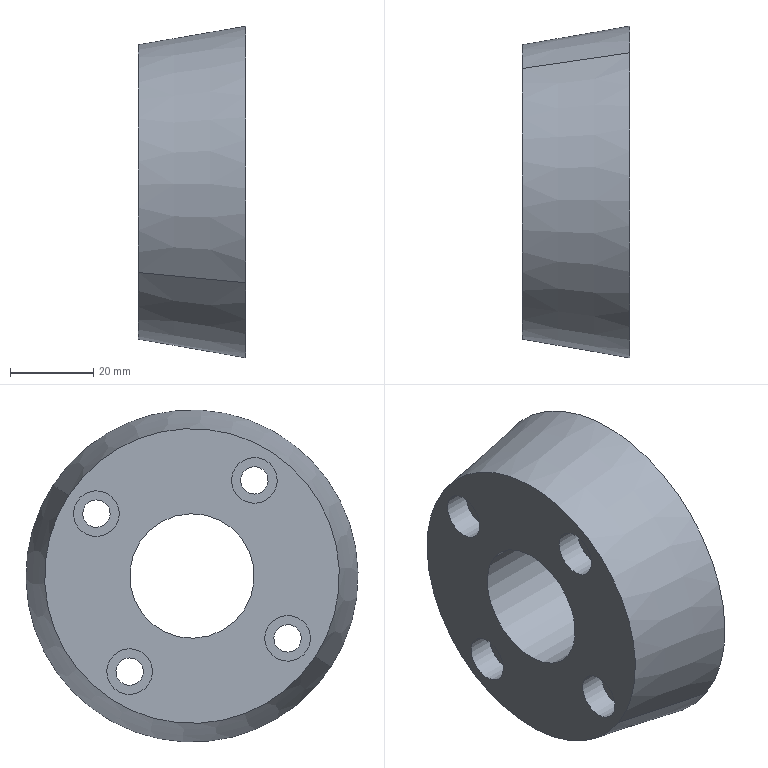Component | SolidWorks | LocatingSleeve3-1_LocatingSleeve3-2-1 | 1 solid | 26 faces | box 26 x 80 x 80 mm | volume 93046 mm3 | cylinder 18 | plane 6 | cone 2 | commonest cylinder face diameters 11 x8 6.6 x8 30 x2
STEP:
#1=CARTESIAN_POINT('',(12.546,-0.9808,30.92));
#2=VERTEX_POINT('',#1);
#3=CARTESIAN_POINT('',(12.546,-0.6181,31.156));
#4=VERTEX_POINT('',#3);
#5=CARTESIAN_POINT('',(12.546,-0.7995,31.038));
#6=DIRECTION('',(-1.,-0.,0.));
#7=DIRECTION('',(0.,0.8375,0.5465));
#8=AXIS2_PLACEMENT_3D('',#5,#6,#7);
#9=CIRCLE('',#8,0.2165);
#10=EDGE_CURVE('',#2,#4,#9,.T.);
#11=ORIENTED_EDGE('',*,*,#10,.F.);
#12=CARTESIAN_POINT('',(12.294,-0.9808,30.92));
#13=VERTEX_POINT('',#12);
#14=CARTESIAN_POINT('',(12.294,-0.9808,30.92));
#15=DIRECTION('',(-1.,-0.,0.));
#16=VECTOR('',#15,39.37);
#17=LINE('',#14,#16);
#18=EDGE_CURVE('',#2,#13,#17,.T.);
#19=ORIENTED_EDGE('',*,*,#18,.T.);
#20=CARTESIAN_POINT('',(12.294,-0.6181,31.156));
#21=VERTEX_POINT('',#20);
#22=CARTESIAN_POINT('',(12.294,-0.7995,31.038));
#23=DIRECTION('',(-1.,-0.,0.));
#24=DIRECTION('',(0.,0.8375,0.5465));
#25=AXIS2_PLACEMENT_3D('',#22,#23,#24);
#26=CIRCLE('',#25,0.2165);
#27=EDGE_CURVE('',#13,#21,#26,.T.);
#28=ORIENTED_EDGE('',*,*,#27,.T.);
#29=CARTESIAN_POINT('',(12.294,-0.6181,31.156));
#30=DIRECTION('',(-1.,-0.,0.));
#31=VECTOR('',#30,39.37);
#32=LINE('',#29,#31);
#33=EDGE_CURVE('',#4,#21,#32,.T.);
#34=ORIENTED_EDGE('',*,*,#33,.F.);
#35=EDGE_LOOP('',(#11,#19,#28,#34));
#36=FACE_OUTER_BOUND('',#35,.T.);
#37=CARTESIAN_POINT('',(12.294,-0.7995,31.038));
#38=DIRECTION('',(-1.,-0.,0.));
#39=DIRECTION('',(0.,0.8375,0.5465));
#40=AXIS2_PLACEMENT_3D('',#37,#38,#39);
#41=CYLINDRICAL_SURFACE('',#40,0.2165);
#42=ADVANCED_FACE('',(#36),#41,.F.);
#43=CARTESIAN_POINT('',(13.318,-0.9083,30.967));
#44=VERTEX_POINT('',#43);
#45=CARTESIAN_POINT('',(13.318,-0.6907,31.109));
#46=VERTEX_POINT('',#45);
#47=CARTESIAN_POINT('',(13.318,-0.7995,31.038));
#48=DIRECTION('',(-1.,-0.,0.));
#49=DIRECTION('',(0.,0.8375,0.5465));
#50=AXIS2_PLACEMENT_3D('',#47,#48,#49);
#51=CIRCLE('',#50,0.1299);
#52=EDGE_CURVE('',#44,#46,#51,.T.);
#53=ORIENTED_EDGE('',*,*,#52,.F.);
#54=CARTESIAN_POINT('',(12.546,-0.9083,30.967));
#55=VERTEX_POINT('',#54);
#56=CARTESIAN_POINT('',(12.294,-0.9083,30.967));
#57=DIRECTION('',(-1.,-0.,0.));
#58=VECTOR('',#57,39.37);
#59=LINE('',#56,#58);
#60=EDGE_CURVE('',#44,#55,#59,.T.);
#61=ORIENTED_EDGE('',*,*,#60,.T.);
#62=CARTESIAN_POINT('',(12.546,-0.6907,31.109));
#63=VERTEX_POINT('',#62);
#64=CARTESIAN_POINT('',(12.546,-0.7995,31.038));
#65=DIRECTION('',(-1.,-0.,0.));
#66=DIRECTION('',(0.,0.8375,0.5465));
#67=AXIS2_PLACEMENT_3D('',#64,#65,#66);
#68=CIRCLE('',#67,0.1299);
#69=EDGE_CURVE('',#55,#63,#68,.T.);
#70=ORIENTED_EDGE('',*,*,#69,.T.);
#71=CARTESIAN_POINT('',(12.294,-0.6907,31.109));
#72=DIRECTION('',(-1.,-0.,0.));
#73=VECTOR('',#72,39.37);
#74=LINE('',#71,#73);
#75=EDGE_CURVE('',#46,#63,#74,.T.);
#76=ORIENTED_EDGE('',*,*,#75,.F.);
#77=EDGE_LOOP('',(#53,#61,#70,#76));
#78=FACE_OUTER_BOUND('',#77,.T.);
#79=CARTESIAN_POINT('',(12.294,-0.7995,31.038));
#80=DIRECTION('',(-1.,-0.,0.));
#81=DIRECTION('',(0.,0.8375,0.5465));
#82=AXIS2_PLACEMENT_3D('',#79,#80,#81);
#83=CYLINDRICAL_SURFACE('',#82,0.1299);
#84=ADVANCED_FACE('',(#78),#83,.F.);
#85=CARTESIAN_POINT('',(12.546,-0.6657,32.418));
#86=VERTEX_POINT('',#85);
#87=CARTESIAN_POINT('',(12.546,-0.303,32.655));
#88=VERTEX_POINT('',#87);
#89=CARTESIAN_POINT('',(12.546,-0.4844,32.536));
#90=DIRECTION('',(-1.,-0.,0.));
#91=DIRECTION('',(0.,0.8375,0.5465));
#92=AXIS2_PLACEMENT_3D('',#89,#90,#91);
#93=CIRCLE('',#92,0.2165);
#94=EDGE_CURVE('',#86,#88,#93,.T.);
#95=ORIENTED_EDGE('',*,*,#94,.F.);
#96=CARTESIAN_POINT('',(12.294,-0.6657,32.418));
#97=VERTEX_POINT('',#96);
#98=CARTESIAN_POINT('',(12.294,-0.6657,32.418));
#99=DIRECTION('',(-1.,-0.,0.));
#100=VECTOR('',#99,39.37);
#101=LINE('',#98,#100);
#102=EDGE_CURVE('',#86,#97,#101,.T.);
#103=ORIENTED_EDGE('',*,*,#102,.T.);
#104=CARTESIAN_POINT('',(12.294,-0.303,32.655));
#105=VERTEX_POINT('',#104);
#106=CARTESIAN_POINT('',(12.294,-0.4844,32.536));
#107=DIRECTION('',(-1.,-0.,0.));
#108=DIRECTION('',(0.,0.8375,0.5465));
#109=AXIS2_PLACEMENT_3D('',#106,#107,#108);
#110=CIRCLE('',#109,0.2165);
#111=EDGE_CURVE('',#97,#105,#110,.T.);
#112=ORIENTED_EDGE('',*,*,#111,.T.);
#113=CARTESIAN_POINT('',(12.294,-0.303,32.655));
#114=DIRECTION('',(-1.,-0.,0.));
#115=VECTOR('',#114,39.37);
#116=LINE('',#113,#115);
#117=EDGE_CURVE('',#88,#105,#116,.T.);
#118=ORIENTED_EDGE('',*,*,#117,.F.);
#119=EDGE_LOOP('',(#95,#103,#112,#118));
#120=FACE_OUTER_BOUND('',#119,.T.);
#121=CARTESIAN_POINT('',(12.294,-0.4844,32.536));
#122=DIRECTION('',(-1.,-0.,0.));
#123=DIRECTION('',(0.,0.8375,0.5465));
#124=AXIS2_PLACEMENT_3D('',#121,#122,#123);
#125=CYLINDRICAL_SURFACE('',#124,0.2165);
#126=ADVANCED_FACE('',(#120),#125,.F.);
#127=CARTESIAN_POINT('',(13.318,-0.5932,32.465));
#128=VERTEX_POINT('',#127);
#129=CARTESIAN_POINT('',(13.318,-0.3756,32.607));
#130=VERTEX_POINT('',#129);
#131=CARTESIAN_POINT('',(13.318,-0.4844,32.536));
#132=DIRECTION('',(-1.,-0.,0.));
#133=DIRECTION('',(0.,0.8375,0.5465));
#134=AXIS2_PLACEMENT_3D('',#131,#132,#133);
#135=CIRCLE('',#134,0.1299);
#136=EDGE_CURVE('',#128,#130,#135,.T.);
#137=ORIENTED_EDGE('',*,*,#136,.F.);
#138=CARTESIAN_POINT('',(12.546,-0.5932,32.465));
#139=VERTEX_POINT('',#138);
#140=CARTESIAN_POINT('',(12.294,-0.5932,32.465));
#141=DIRECTION('',(-1.,-0.,0.));
#142=VECTOR('',#141,39.37);
#143=LINE('',#140,#142);
#144=EDGE_CURVE('',#128,#139,#143,.T.);
#145=ORIENTED_EDGE('',*,*,#144,.T.);
#146=CARTESIAN_POINT('',(12.546,-0.3756,32.607));
#147=VERTEX_POINT('',#146);
#148=CARTESIAN_POINT('',(12.546,-0.4844,32.536));
#149=DIRECTION('',(-1.,-0.,0.));
#150=DIRECTION('',(0.,0.8375,0.5465));
#151=AXIS2_PLACEMENT_3D('',#148,#149,#150);
#152=CIRCLE('',#151,0.1299);
#153=EDGE_CURVE('',#139,#147,#152,.T.);
#154=ORIENTED_EDGE('',*,*,#153,.T.);
#155=CARTESIAN_POINT('',(12.294,-0.3756,32.607));
#156=DIRECTION('',(-1.,-0.,0.));
#157=VECTOR('',#156,39.37);
#158=LINE('',#155,#157);
#159=EDGE_CURVE('',#130,#147,#158,.T.);
#160=ORIENTED_EDGE('',*,*,#159,.F.);
#161=EDGE_LOOP('',(#137,#145,#154,#160));
#162=FACE_OUTER_BOUND('',#161,.T.);
#163=CARTESIAN_POINT('',(12.294,-0.4844,32.536));
#164=DIRECTION('',(-1.,-0.,0.));
#165=DIRECTION('',(0.,0.8375,0.5465));
#166=AXIS2_PLACEMENT_3D('',#163,#164,#165);
#167=CYLINDRICAL_SURFACE('',#166,0.1299);
#168=ADVANCED_FACE('',(#162),#167,.F.);
#169=CARTESIAN_POINT('',(12.546,-2.164,32.733));
#170=VERTEX_POINT('',#169);
#171=CARTESIAN_POINT('',(12.546,-1.801,32.97));
#172=VERTEX_POINT('',#171);
#173=CARTESIAN_POINT('',(12.546,-1.983,32.852));
#174=DIRECTION('',(-1.,-0.,0.));
#175=DIRECTION('',(0.,0.8375,0.5465));
#176=AXIS2_PLACEMENT_3D('',#173,#174,#175);
#177=CIRCLE('',#176,0.2165);
#178=EDGE_CURVE('',#170,#172,#177,.T.);
#179=ORIENTED_EDGE('',*,*,#178,.F.);
#180=CARTESIAN_POINT('',(12.294,-2.164,32.733));
#181=VERTEX_POINT('',#180);
#182=CARTESIAN_POINT('',(12.294,-2.164,32.733));
#183=DIRECTION('',(-1.,-0.,0.));
#184=VECTOR('',#183,39.37);
#185=LINE('',#182,#184);
#186=EDGE_CURVE('',#170,#181,#185,.T.);
#187=ORIENTED_EDGE('',*,*,#186,.T.);
#188=CARTESIAN_POINT('',(12.294,-1.801,32.97));
#189=VERTEX_POINT('',#188);
#190=CARTESIAN_POINT('',(12.294,-1.983,32.852));
#191=DIRECTION('',(-1.,-0.,0.));
#192=DIRECTION('',(0.,0.8375,0.5465));
#193=AXIS2_PLACEMENT_3D('',#190,#191,#192);
#194=CIRCLE('',#193,0.2165);
#195=EDGE_CURVE('',#181,#189,#194,.T.);
#196=ORIENTED_EDGE('',*,*,#195,.T.);
#197=CARTESIAN_POINT('',(12.294,-1.801,32.97));
#198=DIRECTION('',(-1.,-0.,0.));
#199=VECTOR('',#198,39.37);
#200=LINE('',#197,#199);
#201=EDGE_CURVE('',#172,#189,#200,.T.);
#202=ORIENTED_EDGE('',*,*,#201,.F.);
#203=EDGE_LOOP('',(#179,#187,#196,#202));
#204=FACE_OUTER_BOUND('',#203,.T.);
#205=CARTESIAN_POINT('',(12.294,-1.983,32.852));
#206=DIRECTION('',(-1.,-0.,0.));
#207=DIRECTION('',(0.,0.8375,0.5465));
#208=AXIS2_PLACEMENT_3D('',#205,#206,#207);
#209=CYLINDRICAL_SURFACE('',#208,0.2165);
#210=ADVANCED_FACE('',(#204),#209,.F.);
#211=CARTESIAN_POINT('',(13.318,-2.092,32.781));
#212=VERTEX_POINT('',#211);
#213=CARTESIAN_POINT('',(13.318,-1.874,32.923));
#214=VERTEX_POINT('',#213);
#215=CARTESIAN_POINT('',(13.318,-1.983,32.852));
#216=DIRECTION('',(-1.,-0.,0.));
#217=DIRECTION('',(0.,0.8375,0.5465));
#218=AXIS2_PLACEMENT_3D('',#215,#216,#217);
#219=CIRCLE('',#218,0.1299);
#220=EDGE_CURVE('',#212,#214,#219,.T.);
#221=ORIENTED_EDGE('',*,*,#220,.F.);
#222=CARTESIAN_POINT('',(12.546,-2.092,32.781));
#223=VERTEX_POINT('',#222);
#224=CARTESIAN_POINT('',(12.294,-2.092,32.781));
#225=DIRECTION('',(-1.,-0.,0.));
#226=VECTOR('',#225,39.37);
#227=LINE('',#224,#226);
#228=EDGE_CURVE('',#212,#223,#227,.T.);
#229=ORIENTED_EDGE('',*,*,#228,.T.);
#230=CARTESIAN_POINT('',(12.546,-1.874,32.923));
#231=VERTEX_POINT('',#230);
#232=CARTESIAN_POINT('',(12.546,-1.983,32.852));
#233=DIRECTION('',(-1.,-0.,0.));
#234=DIRECTION('',(0.,0.8375,0.5465));
#235=AXIS2_PLACEMENT_3D('',#232,#233,#234);
#236=CIRCLE('',#235,0.1299);
#237=EDGE_CURVE('',#223,#231,#236,.T.);
#238=ORIENTED_EDGE('',*,*,#237,.T.);
#239=CARTESIAN_POINT('',(12.294,-1.874,32.923));
#240=DIRECTION('',(-1.,-0.,0.));
#241=VECTOR('',#240,39.37);
#242=LINE('',#239,#241);
#243=EDGE_CURVE('',#214,#231,#242,.T.);
#244=ORIENTED_EDGE('',*,*,#243,.F.);
#245=EDGE_LOOP('',(#221,#229,#238,#244));
#246=FACE_OUTER_BOUND('',#245,.T.);
#247=CARTESIAN_POINT('',(12.294,-1.983,32.852));
#248=DIRECTION('',(-1.,-0.,0.));
#249=DIRECTION('',(0.,0.8375,0.5465));
#250=AXIS2_PLACEMENT_3D('',#247,#248,#249);
#251=CYLINDRICAL_SURFACE('',#250,0.1299);
#252=ADVANCED_FACE('',(#246),#251,.F.);
#253=CARTESIAN_POINT('',(12.546,-2.479,31.235));
#254=VERTEX_POINT('',#253);
#255=CARTESIAN_POINT('',(12.546,-2.116,31.472));
#256=VERTEX_POINT('',#255);
#257=CARTESIAN_POINT('',(12.546,-2.298,31.353));
#258=DIRECTION('',(-1.,-0.,0.));
#259=DIRECTION('',(0.,0.8375,0.5465));
#260=AXIS2_PLACEMENT_3D('',#257,#258,#259);
#261=CIRCLE('',#260,0.2165);
#262=EDGE_CURVE('',#254,#256,#261,.T.);
#263=ORIENTED_EDGE('',*,*,#262,.F.);
#264=CARTESIAN_POINT('',(12.294,-2.479,31.235));
#265=VERTEX_POINT('',#264);
#266=CARTESIAN_POINT('',(12.294,-2.479,31.235));
#267=DIRECTION('',(-1.,-0.,0.));
#268=VECTOR('',#267,39.37);
#269=LINE('',#266,#268);
#270=EDGE_CURVE('',#254,#265,#269,.T.);
#271=ORIENTED_EDGE('',*,*,#270,.T.);
#272=CARTESIAN_POINT('',(12.294,-2.116,31.472));
#273=VERTEX_POINT('',#272);
#274=CARTESIAN_POINT('',(12.294,-2.298,31.353));
#275=DIRECTION('',(-1.,-0.,0.));
#276=DIRECTION('',(0.,0.8375,0.5465));
#277=AXIS2_PLACEMENT_3D('',#274,#275,#276);
#278=CIRCLE('',#277,0.2165);
#279=EDGE_CURVE('',#265,#273,#278,.T.);
#280=ORIENTED_EDGE('',*,*,#279,.T.);
#281=CARTESIAN_POINT('',(12.294,-2.116,31.472));
#282=DIRECTION('',(-1.,-0.,0.));
#283=VECTOR('',#282,39.37);
#284=LINE('',#281,#283);
#285=EDGE_CURVE('',#256,#273,#284,.T.);
#286=ORIENTED_EDGE('',*,*,#285,.F.);
#287=EDGE_LOOP('',(#263,#271,#280,#286));
#288=FACE_OUTER_BOUND('',#287,.T.);
#289=CARTESIAN_POINT('',(12.294,-2.298,31.353));
#290=DIRECTION('',(-1.,-0.,0.));
#291=DIRECTION('',(0.,0.8375,0.5465));
#292=AXIS2_PLACEMENT_3D('',#289,#290,#291);
#293=CYLINDRICAL_SURFACE('',#292,0.2165);
#294=ADVANCED_FACE('',(#288),#293,.F.);
#295=CARTESIAN_POINT('',(13.318,-2.407,31.282));
#296=VERTEX_POINT('',#295);
#297=CARTESIAN_POINT('',(13.318,-2.189,31.424));
#298=VERTEX_POINT('',#297);
#299=CARTESIAN_POINT('',(13.318,-2.298,31.353));
#300=DIRECTION('',(-1.,-0.,0.));
#301=DIRECTION('',(0.,0.8375,0.5465));
#302=AXIS2_PLACEMENT_3D('',#299,#300,#301);
#303=CIRCLE('',#302,0.1299);
#304=EDGE_CURVE('',#296,#298,#303,.T.);
#305=ORIENTED_EDGE('',*,*,#304,.F.);
#306=CARTESIAN_POINT('',(12.546,-2.407,31.282));
#307=VERTEX_POINT('',#306);
#308=CARTESIAN_POINT('',(12.294,-2.407,31.282));
#309=DIRECTION('',(-1.,-0.,0.));
#310=VECTOR('',#309,39.37);
#311=LINE('',#308,#310);
#312=EDGE_CURVE('',#296,#307,#311,.T.);
#313=ORIENTED_EDGE('',*,*,#312,.T.);
#314=CARTESIAN_POINT('',(12.546,-2.189,31.424));
#315=VERTEX_POINT('',#314);
#316=CARTESIAN_POINT('',(12.546,-2.298,31.353));
#317=DIRECTION('',(-1.,-0.,0.));
#318=DIRECTION('',(0.,0.8375,0.5465));
#319=AXIS2_PLACEMENT_3D('',#316,#317,#318);
#320=CIRCLE('',#319,0.1299);
#321=EDGE_CURVE('',#307,#315,#320,.T.);
#322=ORIENTED_EDGE('',*,*,#321,.T.);
#323=CARTESIAN_POINT('',(12.294,-2.189,31.424));
#324=DIRECTION('',(-1.,-0.,0.));
#325=VECTOR('',#324,39.37);
#326=LINE('',#323,#325);
#327=EDGE_CURVE('',#298,#315,#326,.T.);
#328=ORIENTED_EDGE('',*,*,#327,.F.);
#329=EDGE_LOOP('',(#305,#313,#322,#328));
#330=FACE_OUTER_BOUND('',#329,.T.);
#331=CARTESIAN_POINT('',(12.294,-2.298,31.353));
#332=DIRECTION('',(-1.,-0.,0.));
#333=DIRECTION('',(0.,0.8375,0.5465));
#334=AXIS2_PLACEMENT_3D('',#331,#332,#333);
#335=CYLINDRICAL_SURFACE('',#334,0.1299);
#336=ADVANCED_FACE('',(#330),#335,.F.);
#337=CARTESIAN_POINT('',(12.294,-0.8965,32.268));
#338=VERTEX_POINT('',#337);
#339=CARTESIAN_POINT('',(12.294,-1.886,31.622));
#340=VERTEX_POINT('',#339);
#341=CARTESIAN_POINT('',(12.294,-1.391,31.945));
#342=DIRECTION('',(1.,0.,-0.));
#343=DIRECTION('',(-0.,-0.8375,-0.5465));
#344=AXIS2_PLACEMENT_3D('',#341,#342,#343);
#345=CIRCLE('',#344,0.5906);
#346=EDGE_CURVE('',#338,#340,#345,.T.);
#347=ORIENTED_EDGE('',*,*,#346,.F.);
#348=CARTESIAN_POINT('',(13.318,-0.8965,32.268));
#349=VERTEX_POINT('',#348);
#350=CARTESIAN_POINT('',(13.318,-0.8965,32.268));
#351=DIRECTION('',(1.,0.,-0.));
#352=VECTOR('',#351,39.37);
#353=LINE('',#350,#352);
#354=EDGE_CURVE('',#338,#349,#353,.T.);
#355=ORIENTED_EDGE('',*,*,#354,.T.);
#356=CARTESIAN_POINT('',(13.318,-1.886,31.622));
#357=VERTEX_POINT('',#356);
#358=CARTESIAN_POINT('',(13.318,-1.391,31.945));
#359=DIRECTION('',(1.,0.,-0.));
#360=DIRECTION('',(-0.,-0.8375,-0.5465));
#361=AXIS2_PLACEMENT_3D('',#358,#359,#360);
#362=CIRCLE('',#361,0.5906);
#363=EDGE_CURVE('',#349,#357,#362,.T.);
#364=ORIENTED_EDGE('',*,*,#363,.T.);
#365=CARTESIAN_POINT('',(13.318,-1.886,31.622));
#366=DIRECTION('',(1.,0.,-0.));
#367=VECTOR('',#366,39.37);
#368=LINE('',#365,#367);
#369=EDGE_CURVE('',#340,#357,#368,.T.);
#370=ORIENTED_EDGE('',*,*,#369,.F.);
#371=EDGE_LOOP('',(#347,#355,#364,#370));
#372=FACE_OUTER_BOUND('',#371,.T.);
#373=CARTESIAN_POINT('',(13.318,-1.391,31.945));
#374=DIRECTION('',(1.,0.,-0.));
#375=DIRECTION('',(-0.,-0.8375,-0.5465));
#376=AXIS2_PLACEMENT_3D('',#373,#374,#375);
#377=CYLINDRICAL_SURFACE('',#376,0.5906);
#378=ADVANCED_FACE('',(#372),#377,.F.);
#379=CARTESIAN_POINT('',(12.294,-2.562,31.181));
#380=VERTEX_POINT('',#379);
#381=CARTESIAN_POINT('',(12.294,-0.2206,32.709));
#382=VERTEX_POINT('',#381);
#383=CARTESIAN_POINT('',(12.294,-1.391,31.945));
#384=DIRECTION('',(1.,0.,-0.));
#385=DIRECTION('',(-0.,-0.8375,-0.5465));
#386=AXIS2_PLACEMENT_3D('',#383,#384,#385);
#387=CIRCLE('',#386,1.398);
#388=EDGE_CURVE('',#380,#382,#387,.T.);
#389=ORIENTED_EDGE('',*,*,#388,.T.);
#390=CARTESIAN_POINT('',(13.318,-0.07224,32.805));
#391=VERTEX_POINT('',#390);
#392=CARTESIAN_POINT('',(12.294,-0.2206,32.709));
#393=DIRECTION('',(0.9854,0.1428,0.0932));
#394=VECTOR('',#393,39.37);
#395=LINE('',#392,#394);
#396=EDGE_CURVE('',#382,#391,#395,.T.);
#397=ORIENTED_EDGE('',*,*,#396,.T.);
#398=CARTESIAN_POINT('',(13.318,-2.71,31.084));
#399=VERTEX_POINT('',#398);
#400=CARTESIAN_POINT('',(13.318,-1.391,31.945));
#401=DIRECTION('',(1.,0.,-0.));
#402=DIRECTION('',(-0.,-0.8375,-0.5465));
#403=AXIS2_PLACEMENT_3D('',#400,#401,#402);
#404=CIRCLE('',#403,1.575);
#405=EDGE_CURVE('',#399,#391,#404,.T.);
#406=ORIENTED_EDGE('',*,*,#405,.F.);
#407=CARTESIAN_POINT('',(12.294,-2.562,31.181));
#408=DIRECTION('',(0.9854,-0.1428,-0.0932));
#409=VECTOR('',#408,39.37);
#410=LINE('',#407,#409);
#411=EDGE_CURVE('',#380,#399,#410,.T.);
#412=ORIENTED_EDGE('',*,*,#411,.F.);
#413=EDGE_LOOP('',(#389,#397,#406,#412));
#414=FACE_OUTER_BOUND('',#413,.T.);
#415=CARTESIAN_POINT('',(12.294,-1.391,31.945));
#416=DIRECTION('',(1.,0.,-0.));
#417=DIRECTION('',(-0.,-0.8375,-0.5465));
#418=AXIS2_PLACEMENT_3D('',#415,#416,#417);
#419=CONICAL_SURFACE('',#418,1.398,0.1714);
#420=ADVANCED_FACE('',(#414),#419,.T.);
#421=ORIENTED_EDGE('',*,*,#396,.F.);
#422=CARTESIAN_POINT('',(12.294,-1.391,31.945));
#423=DIRECTION('',(1.,0.,-0.));
#424=DIRECTION('',(-0.,-0.8375,-0.5465));
#425=AXIS2_PLACEMENT_3D('',#422,#423,#424);
#426=CIRCLE('',#425,1.398);
#427=EDGE_CURVE('',#382,#380,#426,.T.);
#428=ORIENTED_EDGE('',*,*,#427,.T.);
#429=ORIENTED_EDGE('',*,*,#411,.T.);
#430=CARTESIAN_POINT('',(13.318,-1.391,31.945));
#431=DIRECTION('',(1.,0.,-0.));
#432=DIRECTION('',(-0.,-0.8375,-0.5465));
#433=AXIS2_PLACEMENT_3D('',#430,#431,#432);
#434=CIRCLE('',#433,1.575);
#435=EDGE_CURVE('',#391,#399,#434,.T.);
#436=ORIENTED_EDGE('',*,*,#435,.F.);
#437=EDGE_LOOP('',(#421,#428,#429,#436));
#438=FACE_OUTER_BOUND('',#437,.T.);
#439=CARTESIAN_POINT('',(12.294,-1.391,31.945));
#440=DIRECTION('',(1.,0.,-0.));
#441=DIRECTION('',(-0.,-0.8375,-0.5465));
#442=AXIS2_PLACEMENT_3D('',#439,#440,#441);
#443=CONICAL_SURFACE('',#442,1.398,0.1714);
#444=ADVANCED_FACE('',(#438),#443,.T.);
#445=CARTESIAN_POINT('',(12.294,-0.7995,31.038));
#446=DIRECTION('',(-1.,-0.,0.));
#447=DIRECTION('',(0.,0.8375,0.5465));
#448=AXIS2_PLACEMENT_3D('',#445,#446,#447);
#449=CIRCLE('',#448,0.2165);
#450=EDGE_CURVE('',#21,#13,#449,.T.);
#451=ORIENTED_EDGE('',*,*,#450,.F.);
#452=ORIENTED_EDGE('',*,*,#27,.F.);
#453=EDGE_LOOP('',(#451,#452));
#454=FACE_BOUND('',#453,.T.);
#455=CARTESIAN_POINT('',(12.294,-0.4844,32.536));
#456=DIRECTION('',(-1.,-0.,0.));
#457=DIRECTION('',(0.,0.8375,0.5465));
#458=AXIS2_PLACEMENT_3D('',#455,#456,#457);
#459=CIRCLE('',#458,0.2165);
#460=EDGE_CURVE('',#105,#97,#459,.T.);
#461=ORIENTED_EDGE('',*,*,#460,.F.);
#462=ORIENTED_EDGE('',*,*,#111,.F.);
#463=EDGE_LOOP('',(#461,#462));
#464=FACE_BOUND('',#463,.T.);
#465=CARTESIAN_POINT('',(12.294,-1.983,32.852));
#466=DIRECTION('',(-1.,-0.,0.));
#467=DIRECTION('',(0.,0.8375,0.5465));
#468=AXIS2_PLACEMENT_3D('',#465,#466,#467);
#469=CIRCLE('',#468,0.2165);
#470=EDGE_CURVE('',#189,#181,#469,.T.);
#471=ORIENTED_EDGE('',*,*,#470,.F.);
#472=ORIENTED_EDGE('',*,*,#195,.F.);
#473=EDGE_LOOP('',(#471,#472));
#474=FACE_BOUND('',#473,.T.);
#475=CARTESIAN_POINT('',(12.294,-2.298,31.353));
#476=DIRECTION('',(-1.,-0.,0.));
#477=DIRECTION('',(0.,0.8375,0.5465));
#478=AXIS2_PLACEMENT_3D('',#475,#476,#477);
#479=CIRCLE('',#478,0.2165);
#480=EDGE_CURVE('',#273,#265,#479,.T.);
#481=ORIENTED_EDGE('',*,*,#480,.F.);
#482=ORIENTED_EDGE('',*,*,#279,.F.);
#483=EDGE_LOOP('',(#481,#482));
#484=FACE_BOUND('',#483,.T.);
#485=ORIENTED_EDGE('',*,*,#388,.F.);
#486=ORIENTED_EDGE('',*,*,#427,.F.);
#487=EDGE_LOOP('',(#485,#486));
#488=FACE_OUTER_BOUND('',#487,.T.);
#489=CARTESIAN_POINT('',(12.294,-1.391,31.945));
#490=DIRECTION('',(1.,0.,-0.));
#491=DIRECTION('',(-0.,-0.8375,-0.5465));
#492=AXIS2_PLACEMENT_3D('',#489,#490,#491);
#493=CIRCLE('',#492,0.5906);
#494=EDGE_CURVE('',#340,#338,#493,.T.);
#495=ORIENTED_EDGE('',*,*,#494,.T.);
#496=ORIENTED_EDGE('',*,*,#346,.T.);
#497=EDGE_LOOP('',(#495,#496));
#498=FACE_BOUND('',#497,.T.);
#499=CARTESIAN_POINT('',(12.294,-0.6273,30.774));
#500=DIRECTION('',(1.,0.,-0.));
#501=DIRECTION('',(-0.,-0.8375,-0.5465));
#502=AXIS2_PLACEMENT_3D('',#499,#500,#501);
#503=PLANE('',#502);
#504=ADVANCED_FACE('',(#454,#464,#474,#484,#488,#498),#503,.F.);
#505=ORIENTED_EDGE('',*,*,#354,.F.);
#506=ORIENTED_EDGE('',*,*,#494,.F.);
#507=ORIENTED_EDGE('',*,*,#369,.T.);
#508=CARTESIAN_POINT('',(13.318,-1.391,31.945));
#509=DIRECTION('',(1.,0.,-0.));
#510=DIRECTION('',(-0.,-0.8375,-0.5465));
#511=AXIS2_PLACEMENT_3D('',#508,#509,#510);
#512=CIRCLE('',#511,0.5906);
#513=EDGE_CURVE('',#357,#349,#512,.T.);
#514=ORIENTED_EDGE('',*,*,#513,.T.);
#515=EDGE_LOOP('',(#505,#506,#507,#514));
#516=FACE_OUTER_BOUND('',#515,.T.);
#517=CARTESIAN_POINT('',(13.318,-1.391,31.945));
#518=DIRECTION('',(1.,0.,-0.));
#519=DIRECTION('',(-0.,-0.8375,-0.5465));
#520=AXIS2_PLACEMENT_3D('',#517,#518,#519);
#521=CYLINDRICAL_SURFACE('',#520,0.5906);
#522=ADVANCED_FACE('',(#516),#521,.F.);
#523=CARTESIAN_POINT('',(13.318,-0.7995,31.038));
#524=DIRECTION('',(-1.,-0.,0.));
#525=DIRECTION('',(0.,0.8375,0.5465));
#526=AXIS2_PLACEMENT_3D('',#523,#524,#525);
#527=CIRCLE('',#526,0.1299);
#528=EDGE_CURVE('',#46,#44,#527,.T.);
#529=ORIENTED_EDGE('',*,*,#528,.T.);
#530=ORIENTED_EDGE('',*,*,#52,.T.);
#531=EDGE_LOOP('',(#529,#530));
#532=FACE_BOUND('',#531,.T.);
#533=CARTESIAN_POINT('',(13.318,-0.4844,32.536));
#534=DIRECTION('',(-1.,-0.,0.));
#535=DIRECTION('',(0.,0.8375,0.5465));
#536=AXIS2_PLACEMENT_3D('',#533,#534,#535);
#537=CIRCLE('',#536,0.1299);
#538=EDGE_CURVE('',#130,#128,#537,.T.);
#539=ORIENTED_EDGE('',*,*,#538,.T.);
#540=ORIENTED_EDGE('',*,*,#136,.T.);
#541=EDGE_LOOP('',(#539,#540));
#542=FACE_BOUND('',#541,.T.);
#543=CARTESIAN_POINT('',(13.318,-1.983,32.852));
#544=DIRECTION('',(-1.,-0.,0.));
#545=DIRECTION('',(0.,0.8375,0.5465));
#546=AXIS2_PLACEMENT_3D('',#543,#544,#545);
#547=CIRCLE('',#546,0.1299);
#548=EDGE_CURVE('',#214,#212,#547,.T.);
#549=ORIENTED_EDGE('',*,*,#548,.T.);
#550=ORIENTED_EDGE('',*,*,#220,.T.);
#551=EDGE_LOOP('',(#549,#550));
#552=FACE_BOUND('',#551,.T.);
#553=CARTESIAN_POINT('',(13.318,-2.298,31.353));
#554=DIRECTION('',(-1.,-0.,0.));
#555=DIRECTION('',(0.,0.8375,0.5465));
#556=AXIS2_PLACEMENT_3D('',#553,#554,#555);
#557=CIRCLE('',#556,0.1299);
#558=EDGE_CURVE('',#298,#296,#557,.T.);
#559=ORIENTED_EDGE('',*,*,#558,.T.);
#560=ORIENTED_EDGE('',*,*,#304,.T.);
#561=EDGE_LOOP('',(#559,#560));
#562=FACE_BOUND('',#561,.T.);
#563=ORIENTED_EDGE('',*,*,#513,.F.);
#564=ORIENTED_EDGE('',*,*,#363,.F.);
#565=EDGE_LOOP('',(#563,#564));
#566=FACE_BOUND('',#565,.T.);
#567=ORIENTED_EDGE('',*,*,#405,.T.);
#568=ORIENTED_EDGE('',*,*,#435,.T.);
#569=EDGE_LOOP('',(#567,#568));
#570=FACE_OUTER_BOUND('',#569,.T.);
#571=CARTESIAN_POINT('',(13.318,-1.068,31.45));
#572=DIRECTION('',(-1.,-0.,0.));
#573=DIRECTION('',(0.,0.8375,0.5465));
#574=AXIS2_PLACEMENT_3D('',#571,#572,#573);
#575=PLANE('',#574);
#576=ADVANCED_FACE('',(#532,#542,#552,#562,#566,#570),#575,.F.);
#577=ORIENTED_EDGE('',*,*,#312,.F.);
#578=ORIENTED_EDGE('',*,*,#558,.F.);
#579=ORIENTED_EDGE('',*,*,#327,.T.);
#580=CARTESIAN_POINT('',(12.546,-2.298,31.353));
#581=DIRECTION('',(-1.,-0.,0.));
#582=DIRECTION('',(0.,0.8375,0.5465));
#583=AXIS2_PLACEMENT_3D('',#580,#581,#582);
#584=CIRCLE('',#583,0.1299);
#585=EDGE_CURVE('',#315,#307,#584,.T.);
#586=ORIENTED_EDGE('',*,*,#585,.T.);
#587=EDGE_LOOP('',(#577,#578,#579,#586));
#588=FACE_OUTER_BOUND('',#587,.T.);
#589=CARTESIAN_POINT('',(12.294,-2.298,31.353));
#590=DIRECTION('',(-1.,-0.,0.));
#591=DIRECTION('',(0.,0.8375,0.5465));
#592=AXIS2_PLACEMENT_3D('',#589,#590,#591);
#593=CYLINDRICAL_SURFACE('',#592,0.1299);
#594=ADVANCED_FACE('',(#588),#593,.F.);
#595=ORIENTED_EDGE('',*,*,#585,.F.);
#596=ORIENTED_EDGE('',*,*,#321,.F.);
#597=EDGE_LOOP('',(#595,#596));
#598=FACE_BOUND('',#597,.T.);
#599=CARTESIAN_POINT('',(12.546,-2.298,31.353));
#600=DIRECTION('',(-1.,-0.,0.));
#601=DIRECTION('',(0.,0.8375,0.5465));
#602=AXIS2_PLACEMENT_3D('',#599,#600,#601);
#603=CIRCLE('',#602,0.2165);
#604=EDGE_CURVE('',#256,#254,#603,.T.);
#605=ORIENTED_EDGE('',*,*,#604,.T.);
#606=ORIENTED_EDGE('',*,*,#262,.T.);
#607=EDGE_LOOP('',(#605,#606));
#608=FACE_OUTER_BOUND('',#607,.T.);
#609=CARTESIAN_POINT('',(12.546,-2.227,31.244));
#610=DIRECTION('',(1.,0.,-0.));
#611=DIRECTION('',(-0.,-0.8375,-0.5465));
#612=AXIS2_PLACEMENT_3D('',#609,#610,#611);
#613=PLANE('',#612);
#614=ADVANCED_FACE('',(#598,#608),#613,.F.);
#615=ORIENTED_EDGE('',*,*,#270,.F.);
#616=ORIENTED_EDGE('',*,*,#604,.F.);
#617=ORIENTED_EDGE('',*,*,#285,.T.);
#618=ORIENTED_EDGE('',*,*,#480,.T.);
#619=EDGE_LOOP('',(#615,#616,#617,#618));
#620=FACE_OUTER_BOUND('',#619,.T.);
#621=CARTESIAN_POINT('',(12.294,-2.298,31.353));
#622=DIRECTION('',(-1.,-0.,0.));
#623=DIRECTION('',(0.,0.8375,0.5465));
#624=AXIS2_PLACEMENT_3D('',#621,#622,#623);
#625=CYLINDRICAL_SURFACE('',#624,0.2165);
#626=ADVANCED_FACE('',(#620),#625,.F.);
#627=ORIENTED_EDGE('',*,*,#228,.F.);
#628=ORIENTED_EDGE('',*,*,#548,.F.);
#629=ORIENTED_EDGE('',*,*,#243,.T.);
#630=CARTESIAN_POINT('',(12.546,-1.983,32.852));
#631=DIRECTION('',(-1.,-0.,0.));
#632=DIRECTION('',(0.,0.8375,0.5465));
#633=AXIS2_PLACEMENT_3D('',#630,#631,#632);
#634=CIRCLE('',#633,0.1299);
#635=EDGE_CURVE('',#231,#223,#634,.T.);
#636=ORIENTED_EDGE('',*,*,#635,.T.);
#637=EDGE_LOOP('',(#627,#628,#629,#636));
#638=FACE_OUTER_BOUND('',#637,.T.);
#639=CARTESIAN_POINT('',(12.294,-1.983,32.852));
#640=DIRECTION('',(-1.,-0.,0.));
#641=DIRECTION('',(0.,0.8375,0.5465));
#642=AXIS2_PLACEMENT_3D('',#639,#640,#641);
#643=CYLINDRICAL_SURFACE('',#642,0.1299);
#644=ADVANCED_FACE('',(#638),#643,.F.);
#645=ORIENTED_EDGE('',*,*,#635,.F.);
#646=ORIENTED_EDGE('',*,*,#237,.F.);
#647=EDGE_LOOP('',(#645,#646));
#648=FACE_BOUND('',#647,.T.);
#649=CARTESIAN_POINT('',(12.546,-1.983,32.852));
#650=DIRECTION('',(-1.,-0.,0.));
#651=DIRECTION('',(0.,0.8375,0.5465));
#652=AXIS2_PLACEMENT_3D('',#649,#650,#651);
#653=CIRCLE('',#652,0.2165);
#654=EDGE_CURVE('',#172,#170,#653,.T.);
#655=ORIENTED_EDGE('',*,*,#654,.T.);
#656=ORIENTED_EDGE('',*,*,#178,.T.);
#657=EDGE_LOOP('',(#655,#656));
#658=FACE_OUTER_BOUND('',#657,.T.);
#659=CARTESIAN_POINT('',(12.546,-1.912,32.743));
#660=DIRECTION('',(1.,0.,-0.));
#661=DIRECTION('',(-0.,-0.8375,-0.5465));
#662=AXIS2_PLACEMENT_3D('',#659,#660,#661);
#663=PLANE('',#662);
#664=ADVANCED_FACE('',(#648,#658),#663,.F.);
#665=ORIENTED_EDGE('',*,*,#186,.F.);
#666=ORIENTED_EDGE('',*,*,#654,.F.);
#667=ORIENTED_EDGE('',*,*,#201,.T.);
#668=ORIENTED_EDGE('',*,*,#470,.T.);
#669=EDGE_LOOP('',(#665,#666,#667,#668));
#670=FACE_OUTER_BOUND('',#669,.T.);
#671=CARTESIAN_POINT('',(12.294,-1.983,32.852));
#672=DIRECTION('',(-1.,-0.,0.));
#673=DIRECTION('',(0.,0.8375,0.5465));
#674=AXIS2_PLACEMENT_3D('',#671,#672,#673);
#675=CYLINDRICAL_SURFACE('',#674,0.2165);
#676=ADVANCED_FACE('',(#670),#675,.F.);
#677=ORIENTED_EDGE('',*,*,#144,.F.);
#678=ORIENTED_EDGE('',*,*,#538,.F.);
#679=ORIENTED_EDGE('',*,*,#159,.T.);
#680=CARTESIAN_POINT('',(12.546,-0.4844,32.536));
#681=DIRECTION('',(-1.,-0.,0.));
#682=DIRECTION('',(0.,0.8375,0.5465));
#683=AXIS2_PLACEMENT_3D('',#680,#681,#682);
#684=CIRCLE('',#683,0.1299);
#685=EDGE_CURVE('',#147,#139,#684,.T.);
#686=ORIENTED_EDGE('',*,*,#685,.T.);
#687=EDGE_LOOP('',(#677,#678,#679,#686));
#688=FACE_OUTER_BOUND('',#687,.T.);
#689=CARTESIAN_POINT('',(12.294,-0.4844,32.536));
#690=DIRECTION('',(-1.,-0.,0.));
#691=DIRECTION('',(0.,0.8375,0.5465));
#692=AXIS2_PLACEMENT_3D('',#689,#690,#691);
#693=CYLINDRICAL_SURFACE('',#692,0.1299);
#694=ADVANCED_FACE('',(#688),#693,.F.);
#695=ORIENTED_EDGE('',*,*,#685,.F.);
#696=ORIENTED_EDGE('',*,*,#153,.F.);
#697=EDGE_LOOP('',(#695,#696));
#698=FACE_BOUND('',#697,.T.);
#699=CARTESIAN_POINT('',(12.546,-0.4844,32.536));
#700=DIRECTION('',(-1.,-0.,0.));
#701=DIRECTION('',(0.,0.8375,0.5465));
#702=AXIS2_PLACEMENT_3D('',#699,#700,#701);
#703=CIRCLE('',#702,0.2165);
#704=EDGE_CURVE('',#88,#86,#703,.T.);
#705=ORIENTED_EDGE('',*,*,#704,.T.);
#706=ORIENTED_EDGE('',*,*,#94,.T.);
#707=EDGE_LOOP('',(#705,#706));
#708=FACE_OUTER_BOUND('',#707,.T.);
#709=CARTESIAN_POINT('',(12.546,-0.4134,32.428));
#710=DIRECTION('',(1.,0.,-0.));
#711=DIRECTION('',(-0.,-0.8375,-0.5465));
#712=AXIS2_PLACEMENT_3D('',#709,#710,#711);
#713=PLANE('',#712);
#714=ADVANCED_FACE('',(#698,#708),#713,.F.);
#715=ORIENTED_EDGE('',*,*,#102,.F.);
#716=ORIENTED_EDGE('',*,*,#704,.F.);
#717=ORIENTED_EDGE('',*,*,#117,.T.);
#718=ORIENTED_EDGE('',*,*,#460,.T.);
#719=EDGE_LOOP('',(#715,#716,#717,#718));
#720=FACE_OUTER_BOUND('',#719,.T.);
#721=CARTESIAN_POINT('',(12.294,-0.4844,32.536));
#722=DIRECTION('',(-1.,-0.,0.));
#723=DIRECTION('',(0.,0.8375,0.5465));
#724=AXIS2_PLACEMENT_3D('',#721,#722,#723);
#725=CYLINDRICAL_SURFACE('',#724,0.2165);
#726=ADVANCED_FACE('',(#720),#725,.F.);
#727=ORIENTED_EDGE('',*,*,#60,.F.);
#728=ORIENTED_EDGE('',*,*,#528,.F.);
#729=ORIENTED_EDGE('',*,*,#75,.T.);
#730=CARTESIAN_POINT('',(12.546,-0.7995,31.038));
#731=DIRECTION('',(-1.,-0.,0.));
#732=DIRECTION('',(0.,0.8375,0.5465));
#733=AXIS2_PLACEMENT_3D('',#730,#731,#732);
#734=CIRCLE('',#733,0.1299);
#735=EDGE_CURVE('',#63,#55,#734,.T.);
#736=ORIENTED_EDGE('',*,*,#735,.T.);
#737=EDGE_LOOP('',(#727,#728,#729,#736));
#738=FACE_OUTER_BOUND('',#737,.T.);
#739=CARTESIAN_POINT('',(12.294,-0.7995,31.038));
#740=DIRECTION('',(-1.,-0.,0.));
#741=DIRECTION('',(0.,0.8375,0.5465));
#742=AXIS2_PLACEMENT_3D('',#739,#740,#741);
#743=CYLINDRICAL_SURFACE('',#742,0.1299);
#744=ADVANCED_FACE('',(#738),#743,.F.);
#745=ORIENTED_EDGE('',*,*,#735,.F.);
#746=ORIENTED_EDGE('',*,*,#69,.F.);
#747=EDGE_LOOP('',(#745,#746));
#748=FACE_BOUND('',#747,.T.);
#749=CARTESIAN_POINT('',(12.546,-0.7995,31.038));
#750=DIRECTION('',(-1.,-0.,0.));
#751=DIRECTION('',(0.,0.8375,0.5465));
#752=AXIS2_PLACEMENT_3D('',#749,#750,#751);
#753=CIRCLE('',#752,0.2165);
#754=EDGE_CURVE('',#4,#2,#753,.T.);
#755=ORIENTED_EDGE('',*,*,#754,.T.);
#756=ORIENTED_EDGE('',*,*,#10,.T.);
#757=EDGE_LOOP('',(#755,#756));
#758=FACE_OUTER_BOUND('',#757,.T.);
#759=CARTESIAN_POINT('',(12.546,-0.7285,30.929));
#760=DIRECTION('',(1.,0.,-0.));
#761=DIRECTION('',(-0.,-0.8375,-0.5465));
#762=AXIS2_PLACEMENT_3D('',#759,#760,#761);
#763=PLANE('',#762);
#764=ADVANCED_FACE('',(#748,#758),#763,.F.);
#765=ORIENTED_EDGE('',*,*,#18,.F.);
#766=ORIENTED_EDGE('',*,*,#754,.F.);
#767=ORIENTED_EDGE('',*,*,#33,.T.);
#768=ORIENTED_EDGE('',*,*,#450,.T.);
#769=EDGE_LOOP('',(#765,#766,#767,#768));
#770=FACE_OUTER_BOUND('',#769,.T.);
#771=CARTESIAN_POINT('',(12.294,-0.7995,31.038));
#772=DIRECTION('',(-1.,-0.,0.));
#773=DIRECTION('',(0.,0.8375,0.5465));
#774=AXIS2_PLACEMENT_3D('',#771,#772,#773);
#775=CYLINDRICAL_SURFACE('',#774,0.2165);
#776=ADVANCED_FACE('',(#770),#775,.F.);
#777=CLOSED_SHELL('',(#42,#84,#126,#168,#210,#252,#294,#336,#378,#420,#444,#504,#522,#576,#594,#614,#626,#644,#664,#676,#694,#714,#726,#744,#764,#776));
#778=MANIFOLD_SOLID_BREP('',#777);
#779=CARTESIAN_POINT('',(0.,0.,0.));
#780=DIRECTION('',(0.,0.,1.));
#781=DIRECTION('',(1.,0.,0.));
#782=AXIS2_PLACEMENT_3D('',#779,#780,#781);
#783=(LENGTH_UNIT()NAMED_UNIT(*)SI_UNIT($,.METRE.));
#784=LENGTH_MEASURE_WITH_UNIT(LENGTH_MEASURE(0.0254),#783);
#785=DIMENSIONAL_EXPONENTS(1.,0.,0.,0.,0.,0.,0.);
#786=(CONVERSION_BASED_UNIT('',#784)LENGTH_UNIT()NAMED_UNIT(#785));
#787=UNCERTAINTY_MEASURE_WITH_UNIT(LENGTH_MEASURE(0.00001),#786,'','');
#788=(NAMED_UNIT(*)PLANE_ANGLE_UNIT()SI_UNIT($,.RADIAN.));
#789=(NAMED_UNIT(*)SI_UNIT($,.STERADIAN.)SOLID_ANGLE_UNIT());
#790=(GEOMETRIC_REPRESENTATION_CONTEXT(3)GLOBAL_UNCERTAINTY_ASSIGNED_CONTEXT((#787))GLOBAL_UNIT_ASSIGNED_CONTEXT((#786,#788,#789))REPRESENTATION_CONTEXT('',''));
#791=ADVANCED_BREP_SHAPE_REPRESENTATION('',(#778,#782),#790);
#792=COLOUR_RGB('',0.7922,0.8196,0.9333);
#793=FILL_AREA_STYLE_COLOUR('',#792);
#794=FILL_AREA_STYLE('',(#793));
#795=SURFACE_STYLE_FILL_AREA(#794);
#796=SURFACE_SIDE_STYLE('',(#795));
#797=SURFACE_STYLE_USAGE(.BOTH.,#796);
#798=PRESENTATION_STYLE_ASSIGNMENT((#797));
#799=STYLED_ITEM('',(#798),#778);
#800=(LENGTH_UNIT()NAMED_UNIT(*)SI_UNIT($,.METRE.));
#801=LENGTH_MEASURE_WITH_UNIT(LENGTH_MEASURE(0.0254),#800);
#802=DIMENSIONAL_EXPONENTS(1.,0.,0.,0.,0.,0.,0.);
#803=(CONVERSION_BASED_UNIT('',#801)LENGTH_UNIT()NAMED_UNIT(#802));
#804=UNCERTAINTY_MEASURE_WITH_UNIT(LENGTH_MEASURE(0.00001),#803,'','');
#805=(NAMED_UNIT(*)PLANE_ANGLE_UNIT()SI_UNIT($,.RADIAN.));
#806=(NAMED_UNIT(*)SI_UNIT($,.STERADIAN.)SOLID_ANGLE_UNIT());
#807=(GEOMETRIC_REPRESENTATION_CONTEXT(3)GLOBAL_UNCERTAINTY_ASSIGNED_CONTEXT((#804))GLOBAL_UNIT_ASSIGNED_CONTEXT((#803,#805,#806))REPRESENTATION_CONTEXT('',''));
#808=MECHANICAL_DESIGN_GEOMETRIC_PRESENTATION_REPRESENTATION('',(#799),#807);
#809=PRESENTATION_LAYER_ASSIGNMENT('','',(#799));